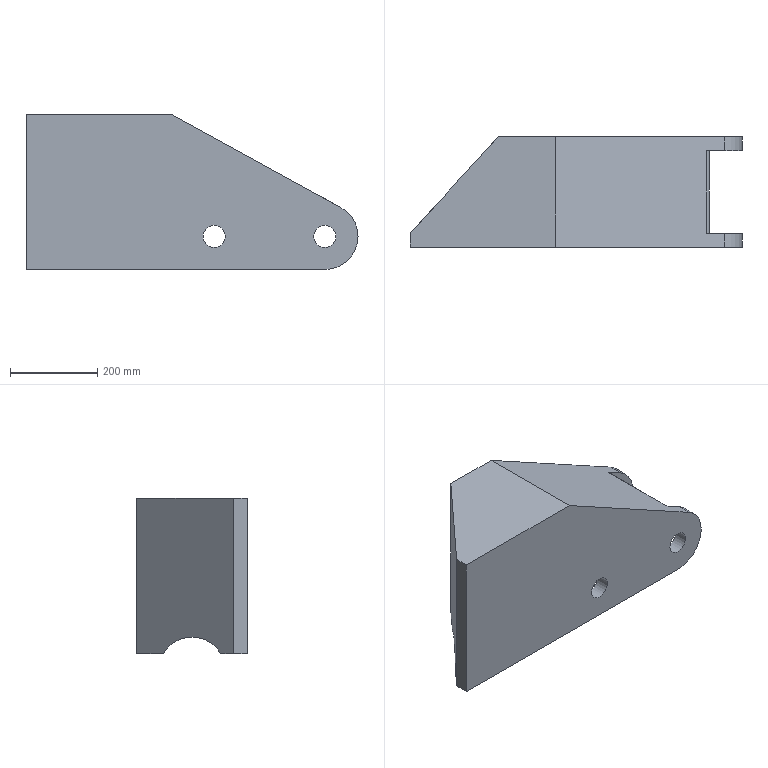Component | NX | CONNECTOR | 1 solid | 27 faces | volume 17956717 mm3 | plane 16 | cylinder 11 | commonest cylinder face diameters 152 x4 50.8 x4 24 x2 152.4 x1